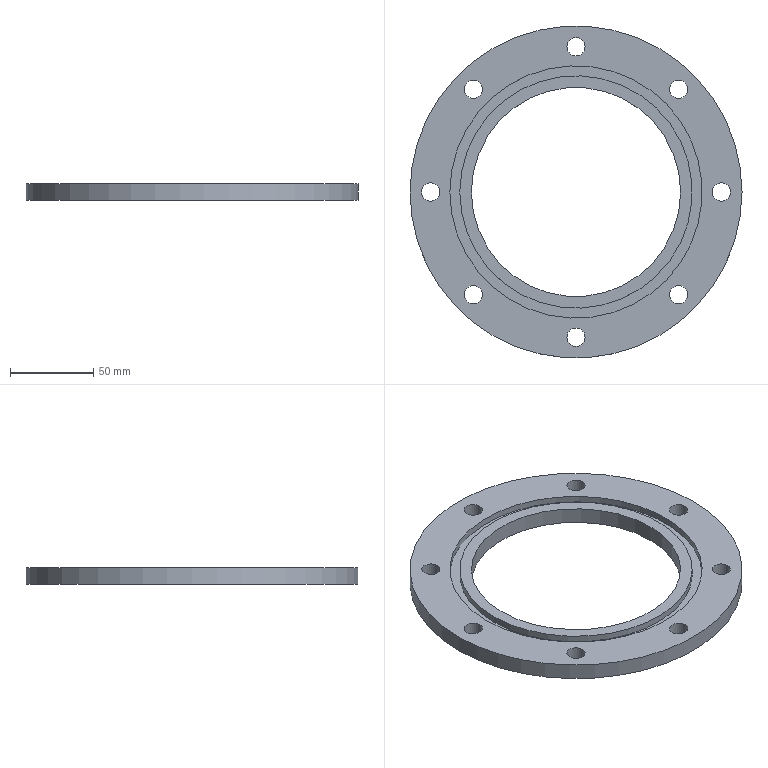Component | NX | CH3404_9-1 | 1 solid | 16 faces | volume 170859 mm3 | cylinder 12 | plane 4 | commonest cylinder face diameters 11 x8 200 x1 126 x1 140 x1 152 x1